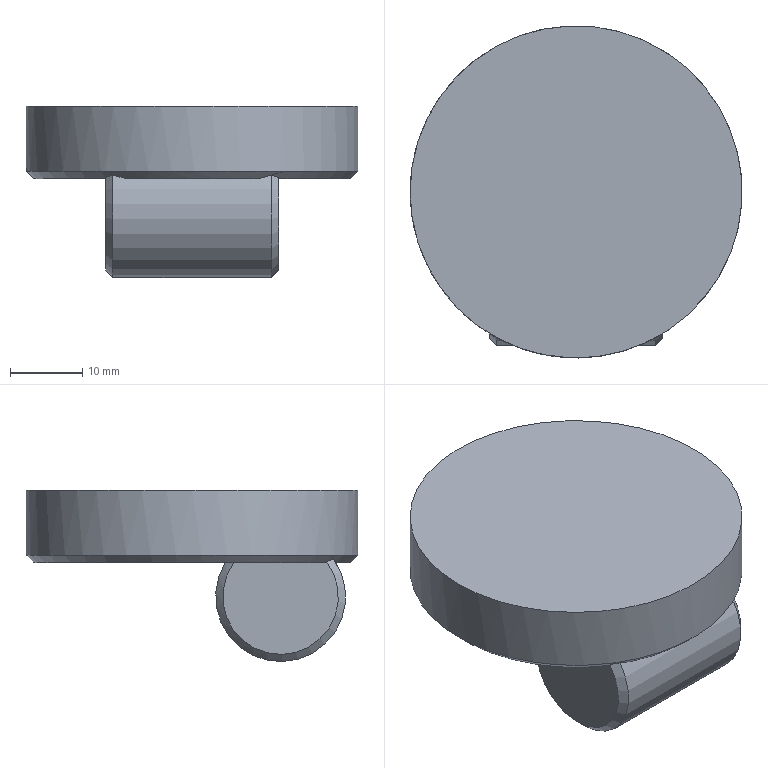Component | NX | FRONT_WHEEL | 1 solid | 11 faces | box 46 x 46 x 23.72 mm | volume 21507 mm3 | plane 5 | cone 4 | cylinder 2 | commonest cylinder face diameters 46 x1 18 x1
STEP:
#1=CARTESIAN_POINT('',(0.,0.,0.));
#2=DIRECTION('',(0.,0.,1.));
#3=DIRECTION('',(1.,0.,0.));
#4=AXIS2_PLACEMENT_3D('',#1,#2,#3);
#5=CARTESIAN_POINT('',(12.615,-161.232,-10.));
#6=VERTEX_POINT('',#5);
#7=CARTESIAN_POINT('',(-12.615,-161.232,-10.));
#8=VERTEX_POINT('',#7);
#9=CARTESIAN_POINT('',(0.,-142.,-10.));
#10=DIRECTION('',(0.,0.,1.));
#11=DIRECTION('',(-1.,0.,0.));
#12=AXIS2_PLACEMENT_3D('',#9,#10,#11);
#13=CIRCLE('',#12,23.);
#14=CARTESIAN_POINT('',(0.,-142.,-11.));
#15=DIRECTION('',(0.,0.,1.));
#16=DIRECTION('',(1.,0.,0.));
#17=AXIS2_PLACEMENT_3D('',#14,#15,#16);
#18=CYLINDRICAL_SURFACE('',#17,23.);
#19=CARTESIAN_POINT('',(3.142,1.));
#20=DIRECTION('',(1.,0.));
#21=VECTOR('',#20,1.);
#22=LINE('',#19,#21);
#23=(GEOMETRIC_REPRESENTATION_CONTEXT(2)PARAMETRIC_REPRESENTATION_CONTEXT()REPRESENTATION_CONTEXT('',''));
#24=DEFINITIONAL_REPRESENTATION('',(#22),#23);
#25=PCURVE('',#18,#24);
#26=CARTESIAN_POINT('',(0.,-142.,-11.));
#27=DIRECTION('',(0.,0.,1.));
#28=DIRECTION('',(1.,0.,0.));
#29=AXIS2_PLACEMENT_3D('',#26,#27,#28);
#30=CONICAL_SURFACE('',#29,22.,0.7854);
#31=CARTESIAN_POINT('',(-3.142,1.));
#32=DIRECTION('',(1.,-0.));
#33=VECTOR('',#32,1.);
#34=LINE('',#31,#33);
#35=(GEOMETRIC_REPRESENTATION_CONTEXT(2)PARAMETRIC_REPRESENTATION_CONTEXT()REPRESENTATION_CONTEXT('',''));
#36=DEFINITIONAL_REPRESENTATION('',(#34),#35);
#37=PCURVE('',#30,#36);
#38=SURFACE_CURVE('',#13,(#25,#37),.PCURVE_S1.);
#39=EDGE_CURVE('',#6,#8,#38,.T.);
#40=ORIENTED_EDGE('',*,*,#39,.T.);
#41=CARTESIAN_POINT('',(-12.545,-161.277,-10.));
#42=VERTEX_POINT('',#41);
#43=CARTESIAN_POINT('',(0.,-142.,-10.));
#44=DIRECTION('',(0.,0.,1.));
#45=DIRECTION('',(-1.,0.,0.));
#46=AXIS2_PLACEMENT_3D('',#43,#44,#45);
#47=CIRCLE('',#46,23.);
#48=CARTESIAN_POINT('',(9.425,1.));
#49=DIRECTION('',(1.,0.));
#50=VECTOR('',#49,1.);
#51=LINE('',#48,#50);
#52=(GEOMETRIC_REPRESENTATION_CONTEXT(2)PARAMETRIC_REPRESENTATION_CONTEXT()REPRESENTATION_CONTEXT('',''));
#53=DEFINITIONAL_REPRESENTATION('',(#51),#52);
#54=PCURVE('',#18,#53);
#55=CARTESIAN_POINT('',(0.,-142.,-11.));
#56=DIRECTION('',(0.,0.,1.));
#57=DIRECTION('',(1.,0.,0.));
#58=AXIS2_PLACEMENT_3D('',#55,#56,#57);
#59=CONICAL_SURFACE('',#58,22.,0.7854);
#60=CARTESIAN_POINT('',(3.142,1.));
#61=DIRECTION('',(1.,-0.));
#62=VECTOR('',#61,1.);
#63=LINE('',#60,#62);
#64=(GEOMETRIC_REPRESENTATION_CONTEXT(2)PARAMETRIC_REPRESENTATION_CONTEXT()REPRESENTATION_CONTEXT('',''));
#65=DEFINITIONAL_REPRESENTATION('',(#63),#64);
#66=PCURVE('',#59,#65);
#67=SURFACE_CURVE('',#47,(#54,#66),.PCURVE_S1.);
#68=EDGE_CURVE('',#8,#42,#67,.T.);
#69=ORIENTED_EDGE('',*,*,#68,.T.);
#70=CARTESIAN_POINT('',(-12.,-161.621,-10.));
#71=VERTEX_POINT('',#70);
#72=CARTESIAN_POINT('',(0.,-142.,-10.));
#73=DIRECTION('',(0.,0.,1.));
#74=DIRECTION('',(-1.,0.,0.));
#75=AXIS2_PLACEMENT_3D('',#72,#73,#74);
#76=CIRCLE('',#75,23.);
#77=CARTESIAN_POINT('',(9.425,1.));
#78=DIRECTION('',(1.,0.));
#79=VECTOR('',#78,1.);
#80=LINE('',#77,#79);
#81=(GEOMETRIC_REPRESENTATION_CONTEXT(2)PARAMETRIC_REPRESENTATION_CONTEXT()REPRESENTATION_CONTEXT('',''));
#82=DEFINITIONAL_REPRESENTATION('',(#80),#81);
#83=PCURVE('',#18,#82);
#84=CARTESIAN_POINT('',(3.142,1.));
#85=DIRECTION('',(1.,-0.));
#86=VECTOR('',#85,1.);
#87=LINE('',#84,#86);
#88=(GEOMETRIC_REPRESENTATION_CONTEXT(2)PARAMETRIC_REPRESENTATION_CONTEXT()REPRESENTATION_CONTEXT('',''));
#89=DEFINITIONAL_REPRESENTATION('',(#87),#88);
#90=PCURVE('',#59,#89);
#91=SURFACE_CURVE('',#76,(#83,#90),.PCURVE_S1.);
#92=EDGE_CURVE('',#42,#71,#91,.T.);
#93=ORIENTED_EDGE('',*,*,#92,.T.);
#94=CARTESIAN_POINT('',(9.702,-162.853,-10.));
#95=VERTEX_POINT('',#94);
#96=CARTESIAN_POINT('',(0.,-142.,-10.));
#97=DIRECTION('',(0.,0.,1.));
#98=DIRECTION('',(-1.,0.,0.));
#99=AXIS2_PLACEMENT_3D('',#96,#97,#98);
#100=CIRCLE('',#99,23.);
#101=CARTESIAN_POINT('',(9.425,1.));
#102=DIRECTION('',(1.,0.));
#103=VECTOR('',#102,1.);
#104=LINE('',#101,#103);
#105=(GEOMETRIC_REPRESENTATION_CONTEXT(2)PARAMETRIC_REPRESENTATION_CONTEXT()REPRESENTATION_CONTEXT('',''));
#106=DEFINITIONAL_REPRESENTATION('',(#104),#105);
#107=PCURVE('',#18,#106);
#108=CARTESIAN_POINT('',(3.142,1.));
#109=DIRECTION('',(1.,0.));
#110=VECTOR('',#109,1.);
#111=LINE('',#108,#110);
#112=(GEOMETRIC_REPRESENTATION_CONTEXT(2)PARAMETRIC_REPRESENTATION_CONTEXT()REPRESENTATION_CONTEXT('',''));
#113=DEFINITIONAL_REPRESENTATION('',(#111),#112);
#114=PCURVE('',#59,#113);
#115=SURFACE_CURVE('',#100,(#107,#114),.PCURVE_S1.);
#116=EDGE_CURVE('',#71,#95,#115,.T.);
#117=ORIENTED_EDGE('',*,*,#116,.T.);
#118=CARTESIAN_POINT('',(12.,-161.621,-10.));
#119=VERTEX_POINT('',#118);
#120=CARTESIAN_POINT('',(0.,-142.,-10.));
#121=DIRECTION('',(0.,0.,1.));
#122=DIRECTION('',(-1.,0.,0.));
#123=AXIS2_PLACEMENT_3D('',#120,#121,#122);
#124=CIRCLE('',#123,23.);
#125=CARTESIAN_POINT('',(9.425,1.));
#126=DIRECTION('',(1.,0.));
#127=VECTOR('',#126,1.);
#128=LINE('',#125,#127);
#129=(GEOMETRIC_REPRESENTATION_CONTEXT(2)PARAMETRIC_REPRESENTATION_CONTEXT()REPRESENTATION_CONTEXT('',''));
#130=DEFINITIONAL_REPRESENTATION('',(#128),#129);
#131=PCURVE('',#18,#130);
#132=CARTESIAN_POINT('',(3.142,1.));
#133=DIRECTION('',(1.,-0.));
#134=VECTOR('',#133,1.);
#135=LINE('',#132,#134);
#136=(GEOMETRIC_REPRESENTATION_CONTEXT(2)PARAMETRIC_REPRESENTATION_CONTEXT()REPRESENTATION_CONTEXT('',''));
#137=DEFINITIONAL_REPRESENTATION('',(#135),#136);
#138=PCURVE('',#59,#137);
#139=SURFACE_CURVE('',#124,(#131,#138),.PCURVE_S1.);
#140=EDGE_CURVE('',#95,#119,#139,.T.);
#141=ORIENTED_EDGE('',*,*,#140,.T.);
#142=CARTESIAN_POINT('',(0.,-142.,-10.));
#143=DIRECTION('',(0.,0.,1.));
#144=DIRECTION('',(-1.,0.,0.));
#145=AXIS2_PLACEMENT_3D('',#142,#143,#144);
#146=CIRCLE('',#145,23.);
#147=CARTESIAN_POINT('',(9.425,1.));
#148=DIRECTION('',(1.,0.));
#149=VECTOR('',#148,1.);
#150=LINE('',#147,#149);
#151=(GEOMETRIC_REPRESENTATION_CONTEXT(2)PARAMETRIC_REPRESENTATION_CONTEXT()REPRESENTATION_CONTEXT('',''));
#152=DEFINITIONAL_REPRESENTATION('',(#150),#151);
#153=PCURVE('',#18,#152);
#154=CARTESIAN_POINT('',(3.142,1.));
#155=DIRECTION('',(1.,0.));
#156=VECTOR('',#155,1.);
#157=LINE('',#154,#156);
#158=(GEOMETRIC_REPRESENTATION_CONTEXT(2)PARAMETRIC_REPRESENTATION_CONTEXT()REPRESENTATION_CONTEXT('',''));
#159=DEFINITIONAL_REPRESENTATION('',(#157),#158);
#160=PCURVE('',#59,#159);
#161=SURFACE_CURVE('',#146,(#153,#160),.PCURVE_S1.);
#162=EDGE_CURVE('',#119,#6,#161,.T.);
#163=ORIENTED_EDGE('',*,*,#162,.T.);
#164=CARTESIAN_POINT('',(12.615,-161.232,-1.));
#165=VERTEX_POINT('',#164);
#166=CARTESIAN_POINT('',(12.615,-161.232,-10.));
#167=CARTESIAN_POINT('',(12.615,-161.232,-1.));
#168=B_SPLINE_CURVE_WITH_KNOTS('',1,(#166,#167),.UNSPECIFIED.,.F.,.F.,(2,2),(1.,10.),.PIECEWISE_BEZIER_KNOTS.);
#169=CARTESIAN_POINT('',(11.576,0.));
#170=DIRECTION('',(0.,1.));
#171=VECTOR('',#170,1.);
#172=LINE('',#169,#171);
#173=(GEOMETRIC_REPRESENTATION_CONTEXT(2)PARAMETRIC_REPRESENTATION_CONTEXT()REPRESENTATION_CONTEXT('',''));
#174=DEFINITIONAL_REPRESENTATION('',(#172),#173);
#175=PCURVE('',#18,#174);
#176=CARTESIAN_POINT('',(5.293,0.));
#177=DIRECTION('',(0.,1.));
#178=VECTOR('',#177,1.);
#179=LINE('',#176,#178);
#180=(GEOMETRIC_REPRESENTATION_CONTEXT(2)PARAMETRIC_REPRESENTATION_CONTEXT()REPRESENTATION_CONTEXT('',''));
#181=DEFINITIONAL_REPRESENTATION('',(#179),#180);
#182=PCURVE('',#18,#181);
#183=SEAM_CURVE('',#168,(#175,#182),.PCURVE_S1.);
#184=EDGE_CURVE('',#6,#165,#183,.T.);
#185=ORIENTED_EDGE('',*,*,#184,.T.);
#186=CARTESIAN_POINT('',(-23.,-142.,-1.));
#187=VERTEX_POINT('',#186);
#188=CARTESIAN_POINT('',(0.,-142.,-1.));
#189=DIRECTION('',(0.,0.,-1.));
#190=DIRECTION('',(-1.,0.,0.));
#191=AXIS2_PLACEMENT_3D('',#188,#189,#190);
#192=CIRCLE('',#191,23.);
#193=CARTESIAN_POINT('',(15.708,10.));
#194=DIRECTION('',(-1.,0.));
#195=VECTOR('',#194,1.);
#196=LINE('',#193,#195);
#197=(GEOMETRIC_REPRESENTATION_CONTEXT(2)PARAMETRIC_REPRESENTATION_CONTEXT()REPRESENTATION_CONTEXT('',''));
#198=DEFINITIONAL_REPRESENTATION('',(#196),#197);
#199=PCURVE('',#18,#198);
#200=CARTESIAN_POINT('',(0.,-142.,-1.));
#201=DIRECTION('',(0.,0.,-1.));
#202=DIRECTION('',(-1.,0.,0.));
#203=AXIS2_PLACEMENT_3D('',#200,#201,#202);
#204=PLANE('',#203);
#205=CARTESIAN_POINT('',(0.,0.));
#206=DIRECTION('',(1.,0.));
#207=AXIS2_PLACEMENT_2D('',#205,#206);
#208=CIRCLE('',#207,23.);
#209=(GEOMETRIC_REPRESENTATION_CONTEXT(2)PARAMETRIC_REPRESENTATION_CONTEXT()REPRESENTATION_CONTEXT('',''));
#210=DEFINITIONAL_REPRESENTATION('',(#208),#209);
#211=PCURVE('',#204,#210);
#212=SURFACE_CURVE('',#192,(#199,#211),.PCURVE_S1.);
#213=EDGE_CURVE('',#165,#187,#212,.T.);
#214=ORIENTED_EDGE('',*,*,#213,.T.);
#215=CARTESIAN_POINT('',(0.,-142.,-1.));
#216=DIRECTION('',(0.,0.,-1.));
#217=DIRECTION('',(-1.,0.,0.));
#218=AXIS2_PLACEMENT_3D('',#215,#216,#217);
#219=CIRCLE('',#218,23.);
#220=CARTESIAN_POINT('',(9.425,10.));
#221=DIRECTION('',(-1.,0.));
#222=VECTOR('',#221,1.);
#223=LINE('',#220,#222);
#224=(GEOMETRIC_REPRESENTATION_CONTEXT(2)PARAMETRIC_REPRESENTATION_CONTEXT()REPRESENTATION_CONTEXT('',''));
#225=DEFINITIONAL_REPRESENTATION('',(#223),#224);
#226=PCURVE('',#18,#225);
#227=CARTESIAN_POINT('',(0.,0.));
#228=DIRECTION('',(1.,0.));
#229=AXIS2_PLACEMENT_2D('',#227,#228);
#230=CIRCLE('',#229,23.);
#231=(GEOMETRIC_REPRESENTATION_CONTEXT(2)PARAMETRIC_REPRESENTATION_CONTEXT()REPRESENTATION_CONTEXT('',''));
#232=DEFINITIONAL_REPRESENTATION('',(#230),#231);
#233=PCURVE('',#204,#232);
#234=SURFACE_CURVE('',#219,(#226,#233),.PCURVE_S1.);
#235=EDGE_CURVE('',#187,#165,#234,.T.);
#236=ORIENTED_EDGE('',*,*,#235,.T.);
#237=ORIENTED_EDGE('',*,*,#184,.F.);
#238=EDGE_LOOP('',(#40,#69,#93,#117,#141,#163,#185,#214,#236,#237));
#239=FACE_BOUND('',#238,.T.);
#240=ADVANCED_FACE('',(#239),#18,.T.);
#241=CARTESIAN_POINT('',(-9.28,-161.947,-11.));
#242=VERTEX_POINT('',#241);
#243=CARTESIAN_POINT('',(9.28,-161.947,-11.));
#244=VERTEX_POINT('',#243);
#245=CARTESIAN_POINT('',(-12.,-161.947,-11.));
#246=DIRECTION('',(1.,0.,0.));
#247=VECTOR('',#246,1.);
#248=LINE('',#245,#247);
#249=CARTESIAN_POINT('',(0.,-142.,-11.));
#250=DIRECTION('',(0.,0.,-1.));
#251=DIRECTION('',(-1.,0.,0.));
#252=AXIS2_PLACEMENT_3D('',#249,#250,#251);
#253=PLANE('',#252);
#254=CARTESIAN_POINT('',(12.,-19.947));
#255=DIRECTION('',(-1.,0.));
#256=VECTOR('',#255,1.);
#257=LINE('',#254,#256);
#258=(GEOMETRIC_REPRESENTATION_CONTEXT(2)PARAMETRIC_REPRESENTATION_CONTEXT()REPRESENTATION_CONTEXT('',''));
#259=DEFINITIONAL_REPRESENTATION('',(#257),#258);
#260=PCURVE('',#253,#259);
#261=CARTESIAN_POINT('',(-12.,-154.286,-15.723));
#262=DIRECTION('',(1.,0.,0.));
#263=DIRECTION('',(0.,0.,-1.));
#264=AXIS2_PLACEMENT_3D('',#261,#262,#263);
#265=CYLINDRICAL_SURFACE('',#264,9.);
#266=CARTESIAN_POINT('',(4.16,0.));
#267=DIRECTION('',(0.,1.));
#268=VECTOR('',#267,1.);
#269=LINE('',#266,#268);
#270=(GEOMETRIC_REPRESENTATION_CONTEXT(2)PARAMETRIC_REPRESENTATION_CONTEXT()REPRESENTATION_CONTEXT('',''));
#271=DEFINITIONAL_REPRESENTATION('',(#269),#270);
#272=PCURVE('',#265,#271);
#273=SURFACE_CURVE('',#248,(#260,#272),.PCURVE_S1.);
#274=EDGE_CURVE('',#242,#244,#273,.T.);
#275=ORIENTED_EDGE('',*,*,#274,.T.);
#276=CARTESIAN_POINT('',(0.,-142.,-11.));
#277=DIRECTION('',(0.,0.,-1.));
#278=DIRECTION('',(-1.,0.,0.));
#279=AXIS2_PLACEMENT_3D('',#276,#277,#278);
#280=CIRCLE('',#279,22.);
#281=CARTESIAN_POINT('',(0.,0.));
#282=DIRECTION('',(1.,0.));
#283=AXIS2_PLACEMENT_2D('',#281,#282);
#284=CIRCLE('',#283,22.);
#285=(GEOMETRIC_REPRESENTATION_CONTEXT(2)PARAMETRIC_REPRESENTATION_CONTEXT()REPRESENTATION_CONTEXT('',''));
#286=DEFINITIONAL_REPRESENTATION('',(#284),#285);
#287=PCURVE('',#253,#286);
#288=CARTESIAN_POINT('',(9.425,0.));
#289=DIRECTION('',(-1.,-0.));
#290=VECTOR('',#289,1.);
#291=LINE('',#288,#290);
#292=(GEOMETRIC_REPRESENTATION_CONTEXT(2)PARAMETRIC_REPRESENTATION_CONTEXT()REPRESENTATION_CONTEXT('',''));
#293=DEFINITIONAL_REPRESENTATION('',(#291),#292);
#294=PCURVE('',#59,#293);
#295=SURFACE_CURVE('',#280,(#287,#294),.PCURVE_S1.);
#296=EDGE_CURVE('',#244,#242,#295,.T.);
#297=ORIENTED_EDGE('',*,*,#296,.T.);
#298=EDGE_LOOP('',(#275,#297));
#299=FACE_BOUND('',#298,.T.);
#300=ADVANCED_FACE('',(#299),#253,.T.);
#301=CARTESIAN_POINT('',(-12.,-160.439,-11.));
#302=VERTEX_POINT('',#301);
#303=CARTESIAN_POINT('',(-12.,-147.829,-11.));
#304=VERTEX_POINT('',#303);
#305=CARTESIAN_POINT('',(-12.,-142.,-11.));
#306=DIRECTION('',(0.,1.,0.));
#307=VECTOR('',#306,1.);
#308=LINE('',#305,#307);
#309=CARTESIAN_POINT('',(0.,-142.,-11.));
#310=DIRECTION('',(0.,0.,-1.));
#311=DIRECTION('',(-1.,0.,0.));
#312=AXIS2_PLACEMENT_3D('',#309,#310,#311);
#313=PLANE('',#312);
#314=CARTESIAN_POINT('',(12.,0.));
#315=DIRECTION('',(0.,1.));
#316=VECTOR('',#315,1.);
#317=LINE('',#314,#316);
#318=(GEOMETRIC_REPRESENTATION_CONTEXT(2)PARAMETRIC_REPRESENTATION_CONTEXT()REPRESENTATION_CONTEXT('',''));
#319=DEFINITIONAL_REPRESENTATION('',(#317),#318);
#320=PCURVE('',#313,#319);
#321=CARTESIAN_POINT('',(-12.,-154.286,-15.723));
#322=DIRECTION('',(-1.,0.,0.));
#323=DIRECTION('',(0.,0.,1.));
#324=AXIS2_PLACEMENT_3D('',#321,#322,#323);
#325=PLANE('',#324);
#326=CARTESIAN_POINT('',(4.723,12.286));
#327=DIRECTION('',(0.,1.));
#328=VECTOR('',#327,1.);
#329=LINE('',#326,#328);
#330=(GEOMETRIC_REPRESENTATION_CONTEXT(2)PARAMETRIC_REPRESENTATION_CONTEXT()REPRESENTATION_CONTEXT('',''));
#331=DEFINITIONAL_REPRESENTATION('',(#329),#330);
#332=PCURVE('',#325,#331);
#333=SURFACE_CURVE('',#308,(#320,#332),.PCURVE_S1.);
#334=EDGE_CURVE('',#302,#304,#333,.T.);
#335=ORIENTED_EDGE('',*,*,#334,.F.);
#336=CARTESIAN_POINT('',(12.,-160.439,-11.));
#337=VERTEX_POINT('',#336);
#338=CARTESIAN_POINT('',(0.,-142.,-11.));
#339=DIRECTION('',(0.,0.,-1.));
#340=DIRECTION('',(-1.,0.,0.));
#341=AXIS2_PLACEMENT_3D('',#338,#339,#340);
#342=CIRCLE('',#341,22.);
#343=CARTESIAN_POINT('',(0.,0.));
#344=DIRECTION('',(1.,0.));
#345=AXIS2_PLACEMENT_2D('',#343,#344);
#346=CIRCLE('',#345,22.);
#347=(GEOMETRIC_REPRESENTATION_CONTEXT(2)PARAMETRIC_REPRESENTATION_CONTEXT()REPRESENTATION_CONTEXT('',''));
#348=DEFINITIONAL_REPRESENTATION('',(#346),#347);
#349=PCURVE('',#313,#348);
#350=CARTESIAN_POINT('',(9.425,0.));
#351=DIRECTION('',(-1.,0.));
#352=VECTOR('',#351,1.);
#353=LINE('',#350,#352);
#354=(GEOMETRIC_REPRESENTATION_CONTEXT(2)PARAMETRIC_REPRESENTATION_CONTEXT()REPRESENTATION_CONTEXT('',''));
#355=DEFINITIONAL_REPRESENTATION('',(#353),#354);
#356=PCURVE('',#30,#355);
#357=SURFACE_CURVE('',#342,(#349,#356),.PCURVE_S1.);
#358=EDGE_CURVE('',#302,#337,#357,.T.);
#359=ORIENTED_EDGE('',*,*,#358,.T.);
#360=CARTESIAN_POINT('',(12.,-147.829,-11.));
#361=VERTEX_POINT('',#360);
#362=CARTESIAN_POINT('',(12.,-142.,-11.));
#363=DIRECTION('',(0.,1.,0.));
#364=VECTOR('',#363,1.);
#365=LINE('',#362,#364);
#366=CARTESIAN_POINT('',(-12.,0.));
#367=DIRECTION('',(0.,1.));
#368=VECTOR('',#367,1.);
#369=LINE('',#366,#368);
#370=(GEOMETRIC_REPRESENTATION_CONTEXT(2)PARAMETRIC_REPRESENTATION_CONTEXT()REPRESENTATION_CONTEXT('',''));
#371=DEFINITIONAL_REPRESENTATION('',(#369),#370);
#372=PCURVE('',#313,#371);
#373=CARTESIAN_POINT('',(12.,-154.286,-15.723));
#374=DIRECTION('',(-1.,0.,0.));
#375=DIRECTION('',(0.,0.,1.));
#376=AXIS2_PLACEMENT_3D('',#373,#374,#375);
#377=PLANE('',#376);
#378=CARTESIAN_POINT('',(4.723,12.286));
#379=DIRECTION('',(0.,1.));
#380=VECTOR('',#379,1.);
#381=LINE('',#378,#380);
#382=(GEOMETRIC_REPRESENTATION_CONTEXT(2)PARAMETRIC_REPRESENTATION_CONTEXT()REPRESENTATION_CONTEXT('',''));
#383=DEFINITIONAL_REPRESENTATION('',(#381),#382);
#384=PCURVE('',#377,#383);
#385=SURFACE_CURVE('',#365,(#372,#384),.PCURVE_S1.);
#386=EDGE_CURVE('',#337,#361,#385,.T.);
#387=ORIENTED_EDGE('',*,*,#386,.T.);
#388=CARTESIAN_POINT('',(11.,-146.625,-11.));
#389=VERTEX_POINT('',#388);
#390=CARTESIAN_POINT('',(12.,-147.829,-11.));
#391=CARTESIAN_POINT('',(11.672,-147.423,-11.));
#392=CARTESIAN_POINT('',(11.338,-147.022,-11.));
#393=CARTESIAN_POINT('',(11.,-146.625,-11.));
#394=B_SPLINE_CURVE_WITH_KNOTS('',3,(#390,#391,#392,#393),.UNSPECIFIED.,.F.,.F.,(4,4),(0.,1.),.PIECEWISE_BEZIER_KNOTS.);
#395=CARTESIAN_POINT('',(-12.,-5.829));
#396=CARTESIAN_POINT('',(-11.672,-5.423));
#397=CARTESIAN_POINT('',(-11.338,-5.022));
#398=CARTESIAN_POINT('',(-11.,-4.625));
#399=B_SPLINE_CURVE_WITH_KNOTS('',3,(#395,#396,#397,#398),.UNSPECIFIED.,.F.,.F.,(4,4),(0.,1.),.PIECEWISE_BEZIER_KNOTS.);
#400=(GEOMETRIC_REPRESENTATION_CONTEXT(2)PARAMETRIC_REPRESENTATION_CONTEXT()REPRESENTATION_CONTEXT('',''));
#401=DEFINITIONAL_REPRESENTATION('',(#399),#400);
#402=PCURVE('',#313,#401);
#403=CARTESIAN_POINT('',(11.,-154.286,-15.723));
#404=DIRECTION('',(-1.,0.,0.));
#405=DIRECTION('',(0.,0.,1.));
#406=AXIS2_PLACEMENT_3D('',#403,#404,#405);
#407=CONICAL_SURFACE('',#406,9.,0.7854);
#408=CARTESIAN_POINT('',(0.9392,-1.));
#409=CARTESIAN_POINT('',(1.018,0.));
#410=B_SPLINE_CURVE_WITH_KNOTS('',1,(#408,#409),.UNSPECIFIED.,.F.,.F.,(2,2),(0.,1.),.PIECEWISE_BEZIER_KNOTS.);
#411=(GEOMETRIC_REPRESENTATION_CONTEXT(2)PARAMETRIC_REPRESENTATION_CONTEXT()REPRESENTATION_CONTEXT('',''));
#412=DEFINITIONAL_REPRESENTATION('',(#410),#411);
#413=PCURVE('',#407,#412);
#414=SURFACE_CURVE('',#394,(#402,#413),.PCURVE_S1.);
#415=EDGE_CURVE('',#361,#389,#414,.T.);
#416=ORIENTED_EDGE('',*,*,#415,.T.);
#417=CARTESIAN_POINT('',(-11.,-146.625,-11.));
#418=VERTEX_POINT('',#417);
#419=CARTESIAN_POINT('',(-12.,-146.625,-11.));
#420=DIRECTION('',(-1.,0.,0.));
#421=VECTOR('',#420,1.);
#422=LINE('',#419,#421);
#423=CARTESIAN_POINT('',(12.,-4.625));
#424=DIRECTION('',(1.,0.));
#425=VECTOR('',#424,1.);
#426=LINE('',#423,#425);
#427=(GEOMETRIC_REPRESENTATION_CONTEXT(2)PARAMETRIC_REPRESENTATION_CONTEXT()REPRESENTATION_CONTEXT('',''));
#428=DEFINITIONAL_REPRESENTATION('',(#426),#427);
#429=PCURVE('',#313,#428);
#430=CARTESIAN_POINT('',(8.406,0.));
#431=DIRECTION('',(0.,-1.));
#432=VECTOR('',#431,1.);
#433=LINE('',#430,#432);
#434=(GEOMETRIC_REPRESENTATION_CONTEXT(2)PARAMETRIC_REPRESENTATION_CONTEXT()REPRESENTATION_CONTEXT('',''));
#435=DEFINITIONAL_REPRESENTATION('',(#433),#434);
#436=PCURVE('',#265,#435);
#437=SURFACE_CURVE('',#422,(#429,#436),.PCURVE_S1.);
#438=EDGE_CURVE('',#389,#418,#437,.T.);
#439=ORIENTED_EDGE('',*,*,#438,.T.);
#440=CARTESIAN_POINT('',(-11.,-146.625,-11.));
#441=CARTESIAN_POINT('',(-11.338,-147.022,-11.));
#442=CARTESIAN_POINT('',(-11.672,-147.423,-11.));
#443=CARTESIAN_POINT('',(-12.,-147.829,-11.));
#444=B_SPLINE_CURVE_WITH_KNOTS('',3,(#440,#441,#442,#443),.UNSPECIFIED.,.F.,.F.,(4,4),(0.,1.),.PIECEWISE_BEZIER_KNOTS.);
#445=CARTESIAN_POINT('',(11.,-4.625));
#446=CARTESIAN_POINT('',(11.338,-5.022));
#447=CARTESIAN_POINT('',(11.672,-5.423));
#448=CARTESIAN_POINT('',(12.,-5.829));
#449=B_SPLINE_CURVE_WITH_KNOTS('',3,(#445,#446,#447,#448),.UNSPECIFIED.,.F.,.F.,(4,4),(0.,1.),.PIECEWISE_BEZIER_KNOTS.);
#450=(GEOMETRIC_REPRESENTATION_CONTEXT(2)PARAMETRIC_REPRESENTATION_CONTEXT()REPRESENTATION_CONTEXT('',''));
#451=DEFINITIONAL_REPRESENTATION('',(#449),#450);
#452=PCURVE('',#313,#451);
#453=CARTESIAN_POINT('',(-12.,-154.286,-15.723));
#454=DIRECTION('',(1.,0.,0.));
#455=DIRECTION('',(0.,0.,-1.));
#456=AXIS2_PLACEMENT_3D('',#453,#454,#455);
#457=CONICAL_SURFACE('',#456,8.,0.7854);
#458=CARTESIAN_POINT('',(8.406,1.));
#459=CARTESIAN_POINT('',(8.486,0.));
#460=B_SPLINE_CURVE_WITH_KNOTS('',1,(#458,#459),.UNSPECIFIED.,.F.,.F.,(2,2),(0.,1.),.PIECEWISE_BEZIER_KNOTS.);
#461=(GEOMETRIC_REPRESENTATION_CONTEXT(2)PARAMETRIC_REPRESENTATION_CONTEXT()REPRESENTATION_CONTEXT('',''));
#462=DEFINITIONAL_REPRESENTATION('',(#460),#461);
#463=PCURVE('',#457,#462);
#464=SURFACE_CURVE('',#444,(#452,#463),.PCURVE_S1.);
#465=EDGE_CURVE('',#418,#304,#464,.T.);
#466=ORIENTED_EDGE('',*,*,#465,.T.);
#467=EDGE_LOOP('',(#335,#359,#387,#416,#439,#466));
#468=FACE_BOUND('',#467,.T.);
#469=ADVANCED_FACE('',(#468),#313,.T.);
#470=ORIENTED_EDGE('',*,*,#235,.F.);
#471=ORIENTED_EDGE('',*,*,#213,.F.);
#472=EDGE_LOOP('',(#470,#471));
#473=FACE_BOUND('',#472,.T.);
#474=ADVANCED_FACE('',(#473),#204,.F.);
#475=ORIENTED_EDGE('',*,*,#334,.T.);
#476=CARTESIAN_POINT('',(-12.,-160.625,-10.844));
#477=VERTEX_POINT('',#476);
#478=CARTESIAN_POINT('',(-12.,-154.286,-15.723));
#479=DIRECTION('',(-1.,0.,0.));
#480=DIRECTION('',(0.,0.,1.));
#481=AXIS2_PLACEMENT_3D('',#478,#479,#480);
#482=CIRCLE('',#481,8.);
#483=CARTESIAN_POINT('',(0.,0.));
#484=DIRECTION('',(1.,0.));
#485=AXIS2_PLACEMENT_2D('',#483,#484);
#486=CIRCLE('',#485,8.);
#487=(GEOMETRIC_REPRESENTATION_CONTEXT(2)PARAMETRIC_REPRESENTATION_CONTEXT()REPRESENTATION_CONTEXT('',''));
#488=DEFINITIONAL_REPRESENTATION('',(#486),#487);
#489=PCURVE('',#325,#488);
#490=CARTESIAN_POINT('',(9.425,0.));
#491=DIRECTION('',(-1.,0.));
#492=VECTOR('',#491,1.);
#493=LINE('',#490,#492);
#494=(GEOMETRIC_REPRESENTATION_CONTEXT(2)PARAMETRIC_REPRESENTATION_CONTEXT()REPRESENTATION_CONTEXT('',''));
#495=DEFINITIONAL_REPRESENTATION('',(#493),#494);
#496=PCURVE('',#457,#495);
#497=SURFACE_CURVE('',#482,(#489,#496),.PCURVE_S1.);
#498=EDGE_CURVE('',#304,#477,#497,.T.);
#499=ORIENTED_EDGE('',*,*,#498,.T.);
#500=CARTESIAN_POINT('',(-12.,-160.625,-10.844));
#501=CARTESIAN_POINT('',(-12.,-160.563,-10.896));
#502=CARTESIAN_POINT('',(-12.,-160.501,-10.948));
#503=CARTESIAN_POINT('',(-12.,-160.439,-11.));
#504=B_SPLINE_CURVE_WITH_KNOTS('',3,(#500,#501,#502,#503),.UNSPECIFIED.,.F.,.F.,(4,4),(0.,1.),.PIECEWISE_BEZIER_KNOTS.);
#505=CARTESIAN_POINT('',(4.88,-6.339));
#506=CARTESIAN_POINT('',(4.828,-6.277));
#507=CARTESIAN_POINT('',(4.776,-6.215));
#508=CARTESIAN_POINT('',(4.723,-6.153));
#509=B_SPLINE_CURVE_WITH_KNOTS('',3,(#505,#506,#507,#508),.UNSPECIFIED.,.F.,.F.,(4,4),(0.,1.),.PIECEWISE_BEZIER_KNOTS.);
#510=(GEOMETRIC_REPRESENTATION_CONTEXT(2)PARAMETRIC_REPRESENTATION_CONTEXT()REPRESENTATION_CONTEXT('',''));
#511=DEFINITIONAL_REPRESENTATION('',(#509),#510);
#512=PCURVE('',#325,#511);
#513=CARTESIAN_POINT('',(4.14,0.1563));
#514=CARTESIAN_POINT('',(4.135,0.));
#515=B_SPLINE_CURVE_WITH_KNOTS('',1,(#513,#514),.UNSPECIFIED.,.F.,.F.,(2,2),(0.,1.),.PIECEWISE_BEZIER_KNOTS.);
#516=(GEOMETRIC_REPRESENTATION_CONTEXT(2)PARAMETRIC_REPRESENTATION_CONTEXT()REPRESENTATION_CONTEXT('',''));
#517=DEFINITIONAL_REPRESENTATION('',(#515),#516);
#518=PCURVE('',#30,#517);
#519=SURFACE_CURVE('',#504,(#512,#518),.PCURVE_S1.);
#520=EDGE_CURVE('',#477,#302,#519,.T.);
#521=ORIENTED_EDGE('',*,*,#520,.T.);
#522=EDGE_LOOP('',(#475,#499,#521));
#523=FACE_BOUND('',#522,.T.);
#524=ADVANCED_FACE('',(#523),#325,.T.);
#525=CARTESIAN_POINT('',(12.,-160.625,-10.844));
#526=VERTEX_POINT('',#525);
#527=CARTESIAN_POINT('',(12.,-160.439,-11.));
#528=CARTESIAN_POINT('',(12.,-160.501,-10.948));
#529=CARTESIAN_POINT('',(12.,-160.563,-10.896));
#530=CARTESIAN_POINT('',(12.,-160.625,-10.844));
#531=B_SPLINE_CURVE_WITH_KNOTS('',3,(#527,#528,#529,#530),.UNSPECIFIED.,.F.,.F.,(4,4),(0.,1.),.PIECEWISE_BEZIER_KNOTS.);
#532=CARTESIAN_POINT('',(4.723,-6.153));
#533=CARTESIAN_POINT('',(4.776,-6.215));
#534=CARTESIAN_POINT('',(4.828,-6.277));
#535=CARTESIAN_POINT('',(4.88,-6.339));
#536=B_SPLINE_CURVE_WITH_KNOTS('',3,(#532,#533,#534,#535),.UNSPECIFIED.,.F.,.F.,(4,4),(0.,1.),.PIECEWISE_BEZIER_KNOTS.);
#537=(GEOMETRIC_REPRESENTATION_CONTEXT(2)PARAMETRIC_REPRESENTATION_CONTEXT()REPRESENTATION_CONTEXT('',''));
#538=DEFINITIONAL_REPRESENTATION('',(#536),#537);
#539=PCURVE('',#377,#538);
#540=CARTESIAN_POINT('',(-0.9939,0.));
#541=CARTESIAN_POINT('',(-0.9984,0.1563));
#542=B_SPLINE_CURVE_WITH_KNOTS('',1,(#540,#541),.UNSPECIFIED.,.F.,.F.,(2,2),(0.,1.),.PIECEWISE_BEZIER_KNOTS.);
#543=(GEOMETRIC_REPRESENTATION_CONTEXT(2)PARAMETRIC_REPRESENTATION_CONTEXT()REPRESENTATION_CONTEXT('',''));
#544=DEFINITIONAL_REPRESENTATION('',(#542),#543);
#545=PCURVE('',#30,#544);
#546=SURFACE_CURVE('',#531,(#539,#545),.PCURVE_S1.);
#547=EDGE_CURVE('',#337,#526,#546,.T.);
#548=ORIENTED_EDGE('',*,*,#547,.T.);
#549=CARTESIAN_POINT('',(12.,-154.286,-15.723));
#550=DIRECTION('',(1.,0.,0.));
#551=DIRECTION('',(0.,0.,1.));
#552=AXIS2_PLACEMENT_3D('',#549,#550,#551);
#553=CIRCLE('',#552,8.);
#554=CARTESIAN_POINT('',(8.,0.));
#555=CARTESIAN_POINT('',(8.,-13.856));
#556=CARTESIAN_POINT('',(-4.,-6.928));
#557=CARTESIAN_POINT('',(-16.,-0.));
#558=CARTESIAN_POINT('',(-4.,6.928));
#559=CARTESIAN_POINT('',(8.,13.856));
#560=CARTESIAN_POINT('',(8.,0.));
#561=(BOUNDED_CURVE()B_SPLINE_CURVE(2,(#554,#555,#556,#557,#558,#559,#560),.UNSPECIFIED.,.T.,.F.)B_SPLINE_CURVE_WITH_KNOTS((1,2,2,2,2,1),(-2.094,0.,2.094,4.189,6.283,8.378),.UNSPECIFIED.)CURVE()GEOMETRIC_REPRESENTATION_ITEM()RATIONAL_B_SPLINE_CURVE((1.,0.5,1.,0.5,1.,0.5,1.))REPRESENTATION_ITEM(''));
#562=(GEOMETRIC_REPRESENTATION_CONTEXT(2)PARAMETRIC_REPRESENTATION_CONTEXT()REPRESENTATION_CONTEXT('',''));
#563=DEFINITIONAL_REPRESENTATION('',(#561),#562);
#564=PCURVE('',#377,#563);
#565=CARTESIAN_POINT('',(6.283,-1.));
#566=DIRECTION('',(-1.,-0.));
#567=VECTOR('',#566,1.);
#568=LINE('',#565,#567);
#569=(GEOMETRIC_REPRESENTATION_CONTEXT(2)PARAMETRIC_REPRESENTATION_CONTEXT()REPRESENTATION_CONTEXT('',''));
#570=DEFINITIONAL_REPRESENTATION('',(#568),#569);
#571=PCURVE('',#407,#570);
#572=SURFACE_CURVE('',#553,(#564,#571),.PCURVE_S1.);
#573=EDGE_CURVE('',#526,#361,#572,.T.);
#574=ORIENTED_EDGE('',*,*,#573,.T.);
#575=ORIENTED_EDGE('',*,*,#386,.F.);
#576=EDGE_LOOP('',(#548,#574,#575));
#577=FACE_BOUND('',#576,.T.);
#578=ADVANCED_FACE('',(#577),#377,.F.);
#579=CARTESIAN_POINT('',(-11.,-161.62,-10.507));
#580=VERTEX_POINT('',#579);
#581=CARTESIAN_POINT('',(-9.28,-161.947,-11.));
#582=CARTESIAN_POINT('',(-9.86,-161.85,-10.843));
#583=CARTESIAN_POINT('',(-10.433,-161.742,-10.678));
#584=CARTESIAN_POINT('',(-11.,-161.62,-10.507));
#585=B_SPLINE_CURVE_WITH_KNOTS('',3,(#581,#582,#583,#584),.UNSPECIFIED.,.F.,.F.,(4,4),(0.,1.),.PIECEWISE_BEZIER_KNOTS.);
#586=CARTESIAN_POINT('',(4.16,2.72));
#587=CARTESIAN_POINT('',(4.094,1.));
#588=B_SPLINE_CURVE_WITH_KNOTS('',1,(#586,#587),.UNSPECIFIED.,.F.,.F.,(2,2),(0.,1.),.PIECEWISE_BEZIER_KNOTS.);
#589=(GEOMETRIC_REPRESENTATION_CONTEXT(2)PARAMETRIC_REPRESENTATION_CONTEXT()REPRESENTATION_CONTEXT('',''));
#590=DEFINITIONAL_REPRESENTATION('',(#588),#589);
#591=PCURVE('',#265,#590);
#592=CARTESIAN_POINT('',(4.277,0.));
#593=CARTESIAN_POINT('',(4.201,0.4931));
#594=B_SPLINE_CURVE_WITH_KNOTS('',1,(#592,#593),.UNSPECIFIED.,.F.,.F.,(2,2),(0.,1.),.PIECEWISE_BEZIER_KNOTS.);
#595=(GEOMETRIC_REPRESENTATION_CONTEXT(2)PARAMETRIC_REPRESENTATION_CONTEXT()REPRESENTATION_CONTEXT('',''));
#596=DEFINITIONAL_REPRESENTATION('',(#594),#595);
#597=PCURVE('',#59,#596);
#598=SURFACE_CURVE('',#585,(#591,#597),.PCURVE_S1.);
#599=EDGE_CURVE('',#242,#580,#598,.T.);
#600=ORIENTED_EDGE('',*,*,#599,.T.);
#601=CARTESIAN_POINT('',(-11.,-154.286,-15.723));
#602=DIRECTION('',(1.,0.,0.));
#603=DIRECTION('',(0.,0.,1.));
#604=AXIS2_PLACEMENT_3D('',#601,#602,#603);
#605=CIRCLE('',#604,9.);
#606=CARTESIAN_POINT('',(3.142,1.));
#607=DIRECTION('',(1.,0.));
#608=VECTOR('',#607,1.);
#609=LINE('',#606,#608);
#610=(GEOMETRIC_REPRESENTATION_CONTEXT(2)PARAMETRIC_REPRESENTATION_CONTEXT()REPRESENTATION_CONTEXT('',''));
#611=DEFINITIONAL_REPRESENTATION('',(#609),#610);
#612=PCURVE('',#265,#611);
#613=CARTESIAN_POINT('',(3.142,1.));
#614=DIRECTION('',(1.,0.));
#615=VECTOR('',#614,1.);
#616=LINE('',#613,#615);
#617=(GEOMETRIC_REPRESENTATION_CONTEXT(2)PARAMETRIC_REPRESENTATION_CONTEXT()REPRESENTATION_CONTEXT('',''));
#618=DEFINITIONAL_REPRESENTATION('',(#616),#617);
#619=PCURVE('',#457,#618);
#620=SURFACE_CURVE('',#605,(#612,#619),.PCURVE_S1.);
#621=EDGE_CURVE('',#580,#418,#620,.T.);
#622=ORIENTED_EDGE('',*,*,#621,.T.);
#623=ORIENTED_EDGE('',*,*,#438,.F.);
#624=CARTESIAN_POINT('',(11.,-161.62,-10.507));
#625=VERTEX_POINT('',#624);
#626=CARTESIAN_POINT('',(11.,-154.286,-15.723));
#627=DIRECTION('',(-1.,0.,0.));
#628=DIRECTION('',(0.,0.,1.));
#629=AXIS2_PLACEMENT_3D('',#626,#627,#628);
#630=CIRCLE('',#629,9.);
#631=CARTESIAN_POINT('',(9.425,23.));
#632=DIRECTION('',(-1.,0.));
#633=VECTOR('',#632,1.);
#634=LINE('',#631,#633);
#635=(GEOMETRIC_REPRESENTATION_CONTEXT(2)PARAMETRIC_REPRESENTATION_CONTEXT()REPRESENTATION_CONTEXT('',''));
#636=DEFINITIONAL_REPRESENTATION('',(#634),#635);
#637=PCURVE('',#265,#636);
#638=CARTESIAN_POINT('',(0.,0.));
#639=DIRECTION('',(1.,-0.));
#640=VECTOR('',#639,1.);
#641=LINE('',#638,#640);
#642=(GEOMETRIC_REPRESENTATION_CONTEXT(2)PARAMETRIC_REPRESENTATION_CONTEXT()REPRESENTATION_CONTEXT('',''));
#643=DEFINITIONAL_REPRESENTATION('',(#641),#642);
#644=PCURVE('',#407,#643);
#645=SURFACE_CURVE('',#630,(#637,#644),.PCURVE_S1.);
#646=EDGE_CURVE('',#389,#625,#645,.T.);
#647=ORIENTED_EDGE('',*,*,#646,.T.);
#648=CARTESIAN_POINT('',(11.,-161.62,-10.507));
#649=CARTESIAN_POINT('',(10.433,-161.742,-10.678));
#650=CARTESIAN_POINT('',(9.86,-161.85,-10.843));
#651=CARTESIAN_POINT('',(9.28,-161.947,-11.));
#652=B_SPLINE_CURVE_WITH_KNOTS('',3,(#648,#649,#650,#651),.UNSPECIFIED.,.F.,.F.,(4,4),(0.,1.),.PIECEWISE_BEZIER_KNOTS.);
#653=CARTESIAN_POINT('',(4.094,23.));
#654=CARTESIAN_POINT('',(4.16,21.28));
#655=B_SPLINE_CURVE_WITH_KNOTS('',1,(#653,#654),.UNSPECIFIED.,.F.,.F.,(2,2),(0.,1.),.PIECEWISE_BEZIER_KNOTS.);
#656=(GEOMETRIC_REPRESENTATION_CONTEXT(2)PARAMETRIC_REPRESENTATION_CONTEXT()REPRESENTATION_CONTEXT('',''));
#657=DEFINITIONAL_REPRESENTATION('',(#655),#656);
#658=PCURVE('',#265,#657);
#659=CARTESIAN_POINT('',(5.223,0.4931));
#660=CARTESIAN_POINT('',(5.148,0.));
#661=B_SPLINE_CURVE_WITH_KNOTS('',1,(#659,#660),.UNSPECIFIED.,.F.,.F.,(2,2),(0.,1.),.PIECEWISE_BEZIER_KNOTS.);
#662=(GEOMETRIC_REPRESENTATION_CONTEXT(2)PARAMETRIC_REPRESENTATION_CONTEXT()REPRESENTATION_CONTEXT('',''));
#663=DEFINITIONAL_REPRESENTATION('',(#661),#662);
#664=PCURVE('',#59,#663);
#665=SURFACE_CURVE('',#652,(#658,#664),.PCURVE_S1.);
#666=EDGE_CURVE('',#625,#244,#665,.T.);
#667=ORIENTED_EDGE('',*,*,#666,.T.);
#668=ORIENTED_EDGE('',*,*,#274,.F.);
#669=EDGE_LOOP('',(#600,#622,#623,#647,#667,#668));
#670=FACE_BOUND('',#669,.T.);
#671=ADVANCED_FACE('',(#670),#265,.T.);
#672=CARTESIAN_POINT('',(-12.615,-161.232,-10.));
#673=CARTESIAN_POINT('',(-12.082,-161.374,-10.173));
#674=CARTESIAN_POINT('',(-11.544,-161.503,-10.343));
#675=CARTESIAN_POINT('',(-11.,-161.62,-10.507));
#676=B_SPLINE_CURVE_WITH_KNOTS('',3,(#672,#673,#674,#675),.UNSPECIFIED.,.F.,.F.,(4,4),(0.,1.),.PIECEWISE_BEZIER_KNOTS.);
#677=CARTESIAN_POINT('',(4.132,1.));
#678=CARTESIAN_POINT('',(4.201,0.4931));
#679=B_SPLINE_CURVE_WITH_KNOTS('',1,(#677,#678),.UNSPECIFIED.,.F.,.F.,(2,2),(0.,1.),.PIECEWISE_BEZIER_KNOTS.);
#680=(GEOMETRIC_REPRESENTATION_CONTEXT(2)PARAMETRIC_REPRESENTATION_CONTEXT()REPRESENTATION_CONTEXT('',''));
#681=DEFINITIONAL_REPRESENTATION('',(#679),#680);
#682=PCURVE('',#30,#681);
#683=CARTESIAN_POINT('',(4.132,1.));
#684=CARTESIAN_POINT('',(4.201,0.4931));
#685=B_SPLINE_CURVE_WITH_KNOTS('',1,(#683,#684),.UNSPECIFIED.,.F.,.F.,(2,2),(0.,1.),.PIECEWISE_BEZIER_KNOTS.);
#686=(GEOMETRIC_REPRESENTATION_CONTEXT(2)PARAMETRIC_REPRESENTATION_CONTEXT()REPRESENTATION_CONTEXT('',''));
#687=DEFINITIONAL_REPRESENTATION('',(#685),#686);
#688=PCURVE('',#59,#687);
#689=SURFACE_CURVE('',#676,(#682,#688),.PCURVE_S1.);
#690=EDGE_CURVE('',#8,#580,#689,.T.);
#691=ORIENTED_EDGE('',*,*,#690,.F.);
#692=ORIENTED_EDGE('',*,*,#39,.F.);
#693=CARTESIAN_POINT('',(11.,-161.62,-10.507));
#694=CARTESIAN_POINT('',(11.544,-161.503,-10.343));
#695=CARTESIAN_POINT('',(12.082,-161.374,-10.173));
#696=CARTESIAN_POINT('',(12.615,-161.232,-10.));
#697=B_SPLINE_CURVE_WITH_KNOTS('',3,(#693,#694,#695,#696),.UNSPECIFIED.,.F.,.F.,(4,4),(0.,1.),.PIECEWISE_BEZIER_KNOTS.);
#698=CARTESIAN_POINT('',(-1.06,0.4931));
#699=CARTESIAN_POINT('',(-0.9902,1.));
#700=B_SPLINE_CURVE_WITH_KNOTS('',1,(#698,#699),.UNSPECIFIED.,.F.,.F.,(2,2),(0.,1.),.PIECEWISE_BEZIER_KNOTS.);
#701=(GEOMETRIC_REPRESENTATION_CONTEXT(2)PARAMETRIC_REPRESENTATION_CONTEXT()REPRESENTATION_CONTEXT('',''));
#702=DEFINITIONAL_REPRESENTATION('',(#700),#701);
#703=PCURVE('',#30,#702);
#704=CARTESIAN_POINT('',(5.223,0.4931));
#705=CARTESIAN_POINT('',(5.293,1.));
#706=B_SPLINE_CURVE_WITH_KNOTS('',1,(#704,#705),.UNSPECIFIED.,.F.,.F.,(2,2),(0.,1.),.PIECEWISE_BEZIER_KNOTS.);
#707=(GEOMETRIC_REPRESENTATION_CONTEXT(2)PARAMETRIC_REPRESENTATION_CONTEXT()REPRESENTATION_CONTEXT('',''));
#708=DEFINITIONAL_REPRESENTATION('',(#706),#707);
#709=PCURVE('',#59,#708);
#710=SURFACE_CURVE('',#697,(#703,#709),.PCURVE_S1.);
#711=EDGE_CURVE('',#625,#6,#710,.T.);
#712=ORIENTED_EDGE('',*,*,#711,.F.);
#713=CARTESIAN_POINT('',(11.,-161.62,-10.507));
#714=CARTESIAN_POINT('',(11.336,-161.294,-10.627));
#715=CARTESIAN_POINT('',(11.669,-160.962,-10.739));
#716=CARTESIAN_POINT('',(12.,-160.625,-10.844));
#717=B_SPLINE_CURVE_WITH_KNOTS('',3,(#713,#714,#715,#716),.UNSPECIFIED.,.F.,.F.,(4,4),(0.,1.),.PIECEWISE_BEZIER_KNOTS.);
#718=CARTESIAN_POINT('',(-1.06,0.4931));
#719=CARTESIAN_POINT('',(-0.9984,0.1563));
#720=B_SPLINE_CURVE_WITH_KNOTS('',1,(#718,#719),.UNSPECIFIED.,.F.,.F.,(2,2),(0.,1.),.PIECEWISE_BEZIER_KNOTS.);
#721=(GEOMETRIC_REPRESENTATION_CONTEXT(2)PARAMETRIC_REPRESENTATION_CONTEXT()REPRESENTATION_CONTEXT('',''));
#722=DEFINITIONAL_REPRESENTATION('',(#720),#721);
#723=PCURVE('',#30,#722);
#724=CARTESIAN_POINT('',(5.331,0.));
#725=CARTESIAN_POINT('',(5.368,-1.));
#726=B_SPLINE_CURVE_WITH_KNOTS('',1,(#724,#725),.UNSPECIFIED.,.F.,.F.,(2,2),(0.,1.),.PIECEWISE_BEZIER_KNOTS.);
#727=(GEOMETRIC_REPRESENTATION_CONTEXT(2)PARAMETRIC_REPRESENTATION_CONTEXT()REPRESENTATION_CONTEXT('',''));
#728=DEFINITIONAL_REPRESENTATION('',(#726),#727);
#729=PCURVE('',#407,#728);
#730=SURFACE_CURVE('',#717,(#723,#729),.PCURVE_S1.);
#731=EDGE_CURVE('',#625,#526,#730,.T.);
#732=ORIENTED_EDGE('',*,*,#731,.T.);
#733=ORIENTED_EDGE('',*,*,#547,.F.);
#734=ORIENTED_EDGE('',*,*,#358,.F.);
#735=ORIENTED_EDGE('',*,*,#520,.F.);
#736=CARTESIAN_POINT('',(-12.,-160.625,-10.844));
#737=CARTESIAN_POINT('',(-11.669,-160.962,-10.739));
#738=CARTESIAN_POINT('',(-11.336,-161.294,-10.627));
#739=CARTESIAN_POINT('',(-11.,-161.62,-10.507));
#740=B_SPLINE_CURVE_WITH_KNOTS('',3,(#736,#737,#738,#739),.UNSPECIFIED.,.F.,.F.,(4,4),(0.,1.),.PIECEWISE_BEZIER_KNOTS.);
#741=CARTESIAN_POINT('',(4.14,0.1563));
#742=CARTESIAN_POINT('',(4.201,0.4931));
#743=B_SPLINE_CURVE_WITH_KNOTS('',1,(#741,#742),.UNSPECIFIED.,.F.,.F.,(2,2),(0.,1.),.PIECEWISE_BEZIER_KNOTS.);
#744=(GEOMETRIC_REPRESENTATION_CONTEXT(2)PARAMETRIC_REPRESENTATION_CONTEXT()REPRESENTATION_CONTEXT('',''));
#745=DEFINITIONAL_REPRESENTATION('',(#743),#744);
#746=PCURVE('',#30,#745);
#747=CARTESIAN_POINT('',(4.056,-0.));
#748=CARTESIAN_POINT('',(4.094,1.));
#749=B_SPLINE_CURVE_WITH_KNOTS('',1,(#747,#748),.UNSPECIFIED.,.F.,.F.,(2,2),(0.,1.),.PIECEWISE_BEZIER_KNOTS.);
#750=(GEOMETRIC_REPRESENTATION_CONTEXT(2)PARAMETRIC_REPRESENTATION_CONTEXT()REPRESENTATION_CONTEXT('',''));
#751=DEFINITIONAL_REPRESENTATION('',(#749),#750);
#752=PCURVE('',#457,#751);
#753=SURFACE_CURVE('',#740,(#746,#752),.PCURVE_S1.);
#754=EDGE_CURVE('',#477,#580,#753,.T.);
#755=ORIENTED_EDGE('',*,*,#754,.T.);
#756=EDGE_LOOP('',(#691,#692,#712,#732,#733,#734,#735,#755));
#757=FACE_BOUND('',#756,.T.);
#758=ADVANCED_FACE('',(#757),#30,.T.);
#759=ORIENTED_EDGE('',*,*,#68,.F.);
#760=ORIENTED_EDGE('',*,*,#690,.T.);
#761=ORIENTED_EDGE('',*,*,#599,.F.);
#762=ORIENTED_EDGE('',*,*,#296,.F.);
#763=ORIENTED_EDGE('',*,*,#666,.F.);
#764=ORIENTED_EDGE('',*,*,#711,.T.);
#765=ORIENTED_EDGE('',*,*,#162,.F.);
#766=ORIENTED_EDGE('',*,*,#140,.F.);
#767=ORIENTED_EDGE('',*,*,#116,.F.);
#768=ORIENTED_EDGE('',*,*,#92,.F.);
#769=EDGE_LOOP('',(#759,#760,#761,#762,#763,#764,#765,#766,#767,#768));
#770=FACE_BOUND('',#769,.T.);
#771=ADVANCED_FACE('',(#770),#59,.T.);
#772=ORIENTED_EDGE('',*,*,#465,.F.);
#773=ORIENTED_EDGE('',*,*,#621,.F.);
#774=ORIENTED_EDGE('',*,*,#754,.F.);
#775=ORIENTED_EDGE('',*,*,#498,.F.);
#776=EDGE_LOOP('',(#772,#773,#774,#775));
#777=FACE_BOUND('',#776,.T.);
#778=ADVANCED_FACE('',(#777),#457,.T.);
#779=ORIENTED_EDGE('',*,*,#415,.F.);
#780=ORIENTED_EDGE('',*,*,#573,.F.);
#781=ORIENTED_EDGE('',*,*,#731,.F.);
#782=ORIENTED_EDGE('',*,*,#646,.F.);
#783=EDGE_LOOP('',(#779,#780,#781,#782));
#784=FACE_BOUND('',#783,.T.);
#785=ADVANCED_FACE('',(#784),#407,.T.);
#786=CLOSED_SHELL('',(#240,#300,#469,#474,#524,#578,#671,#758,#771,#778,#785));
#787=MANIFOLD_SOLID_BREP('',#786);
#788=(LENGTH_UNIT()NAMED_UNIT(*)SI_UNIT(.MILLI.,.METRE.));
#789=UNCERTAINTY_MEASURE_WITH_UNIT(LENGTH_MEASURE(0.01),#788,'','');
#790=(NAMED_UNIT(*)PLANE_ANGLE_UNIT()SI_UNIT($,.RADIAN.));
#791=(NAMED_UNIT(*)SI_UNIT($,.STERADIAN.)SOLID_ANGLE_UNIT());
#792=(GEOMETRIC_REPRESENTATION_CONTEXT(3)GLOBAL_UNCERTAINTY_ASSIGNED_CONTEXT((#789))GLOBAL_UNIT_ASSIGNED_CONTEXT((#788,#790,#791))REPRESENTATION_CONTEXT('',''));
#793=ADVANCED_BREP_SHAPE_REPRESENTATION('',(#4,#787),#792);